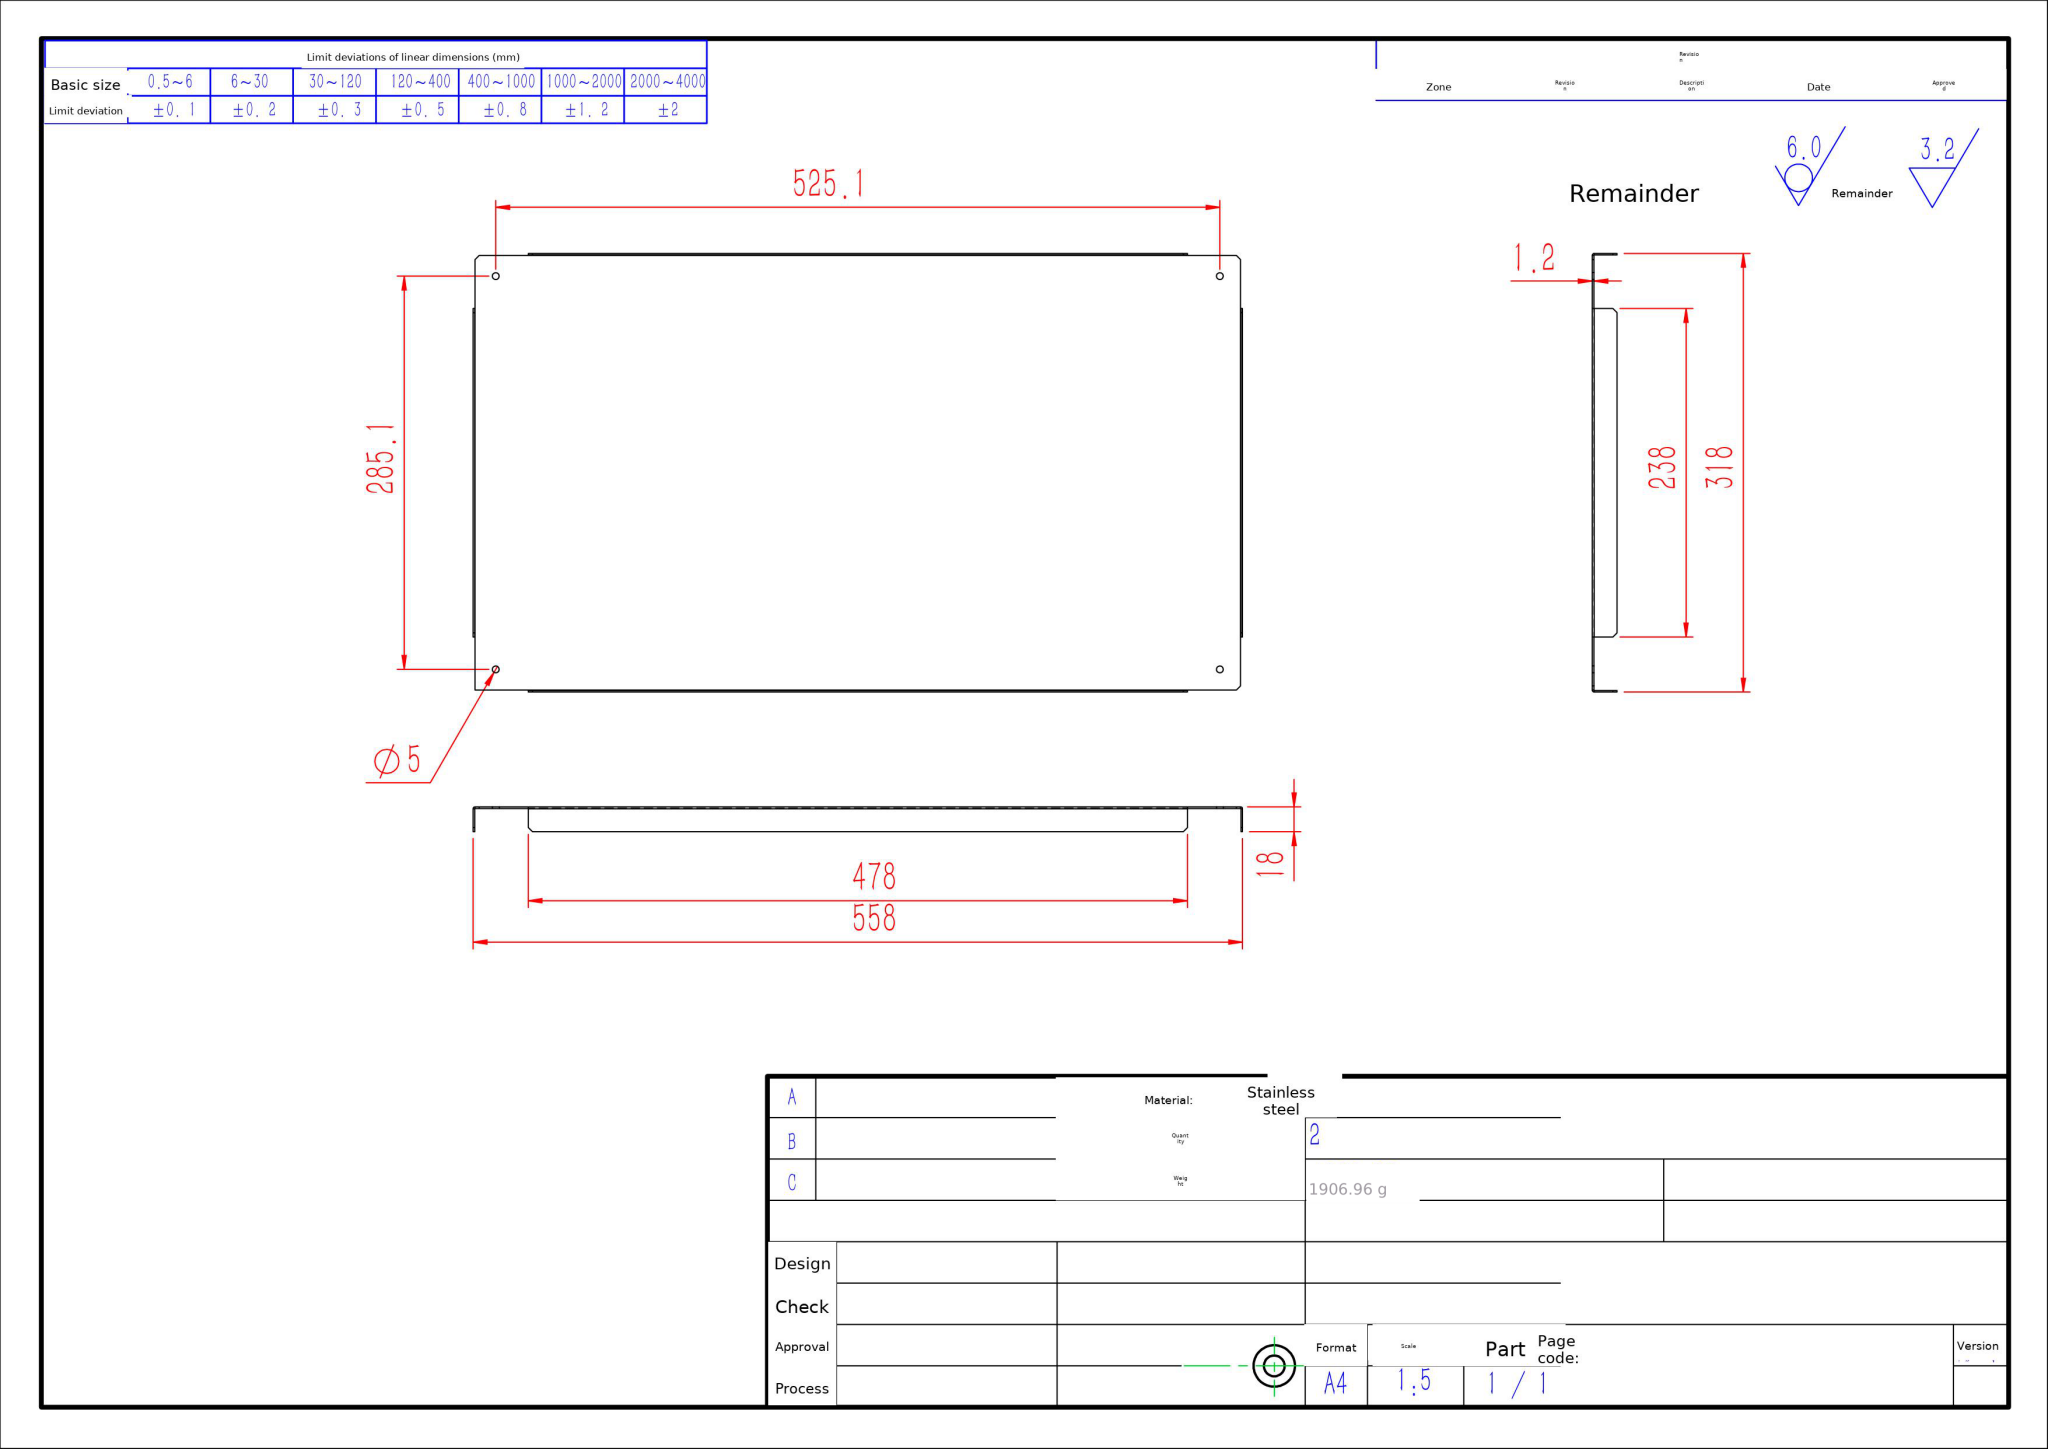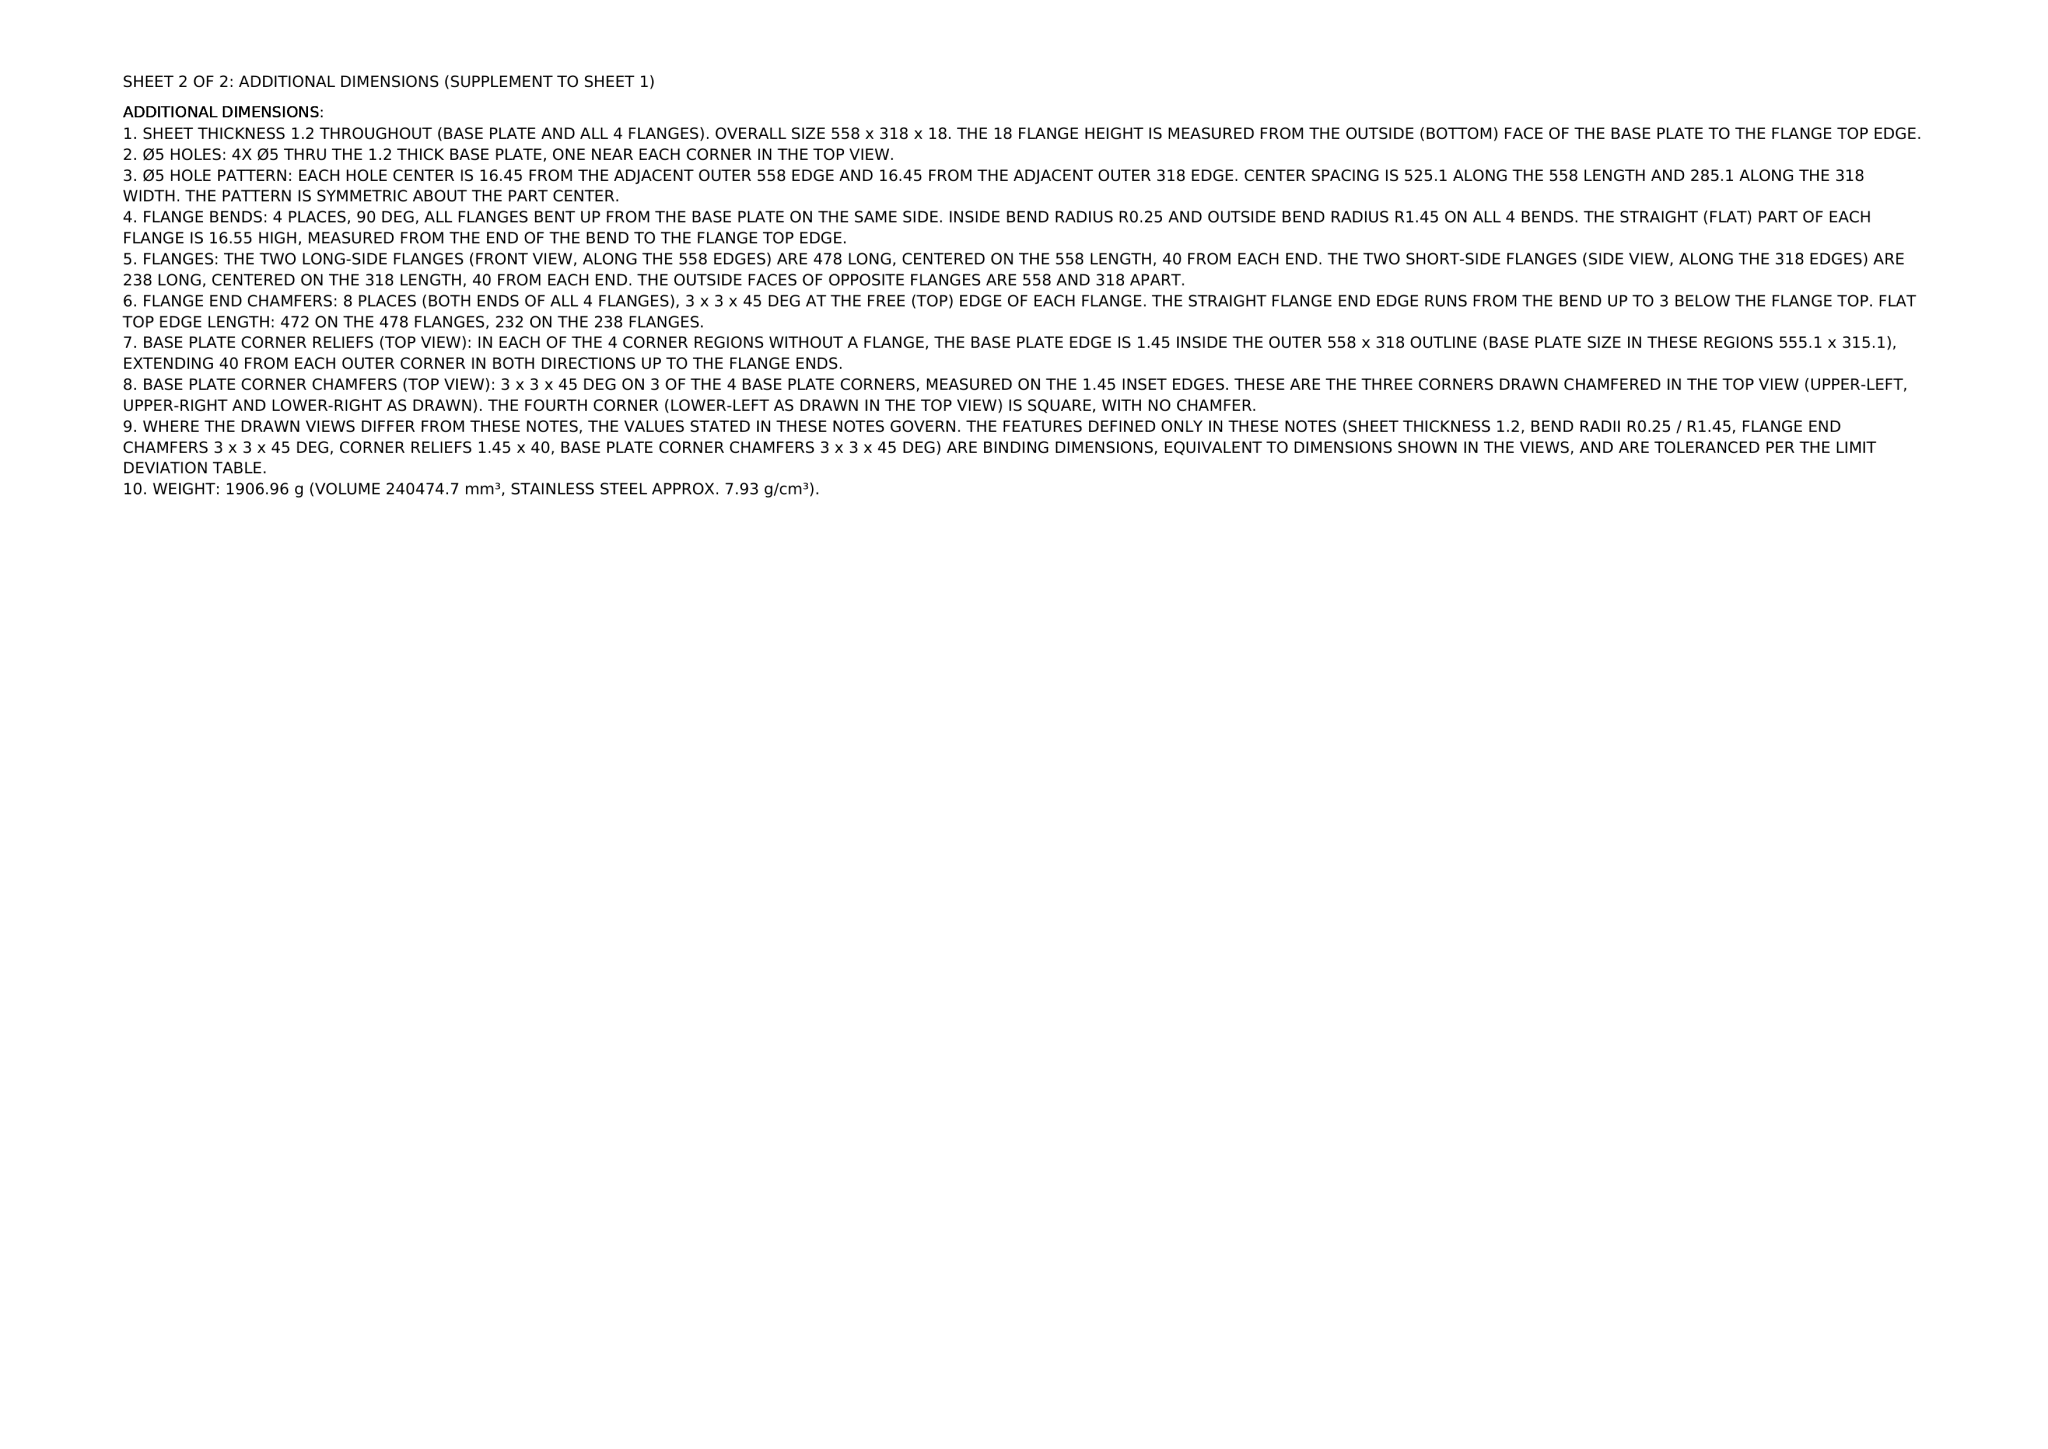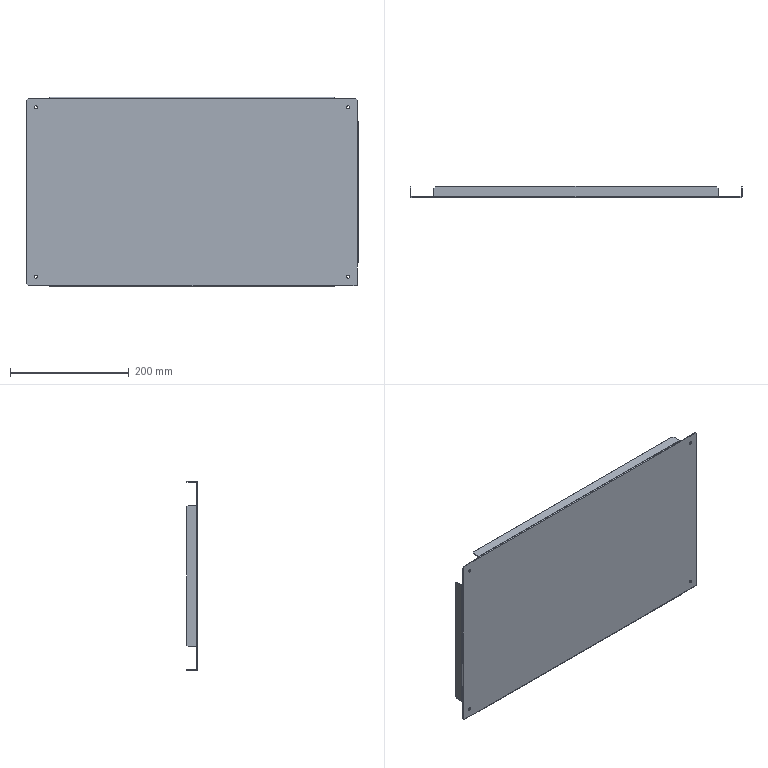Part | NX | mm | 1 solid | 65 faces | box 558 x 18 x 318 mm | volume 240475 mm3 | plane 49 | cylinder 16 | commonest cylinder face diameters 5 x8 2.9 x4 0.5 x4